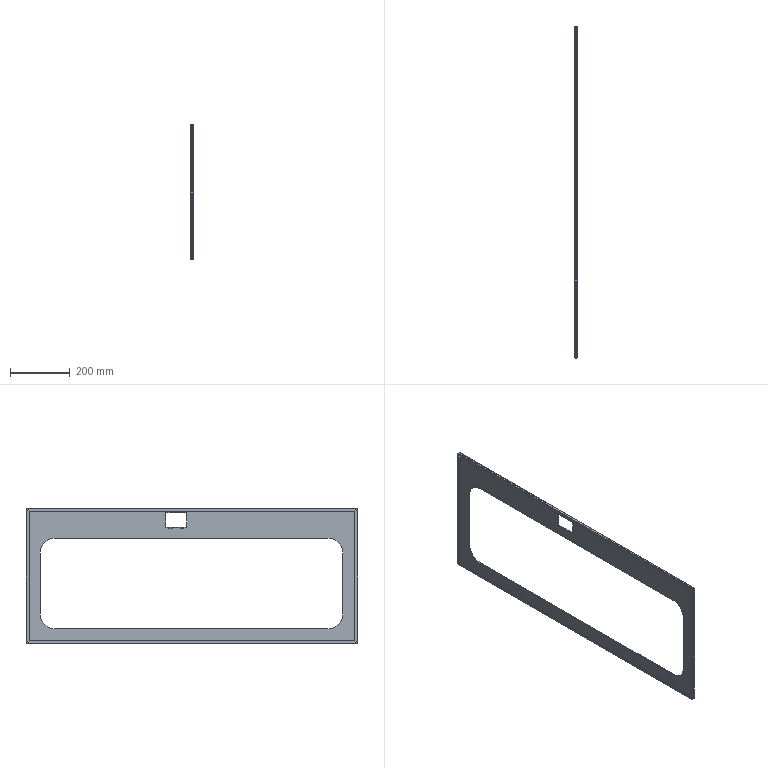Component | SolidWorks | UpperDoorFrame-1_UpperDoor1-3 | 1 solid | 90 faces | volume 363854 mm3 | plane 54 | cylinder 20 | spline 16 | commonest cylinder face diameters 4.473 x8 1.473 x8 100 x4